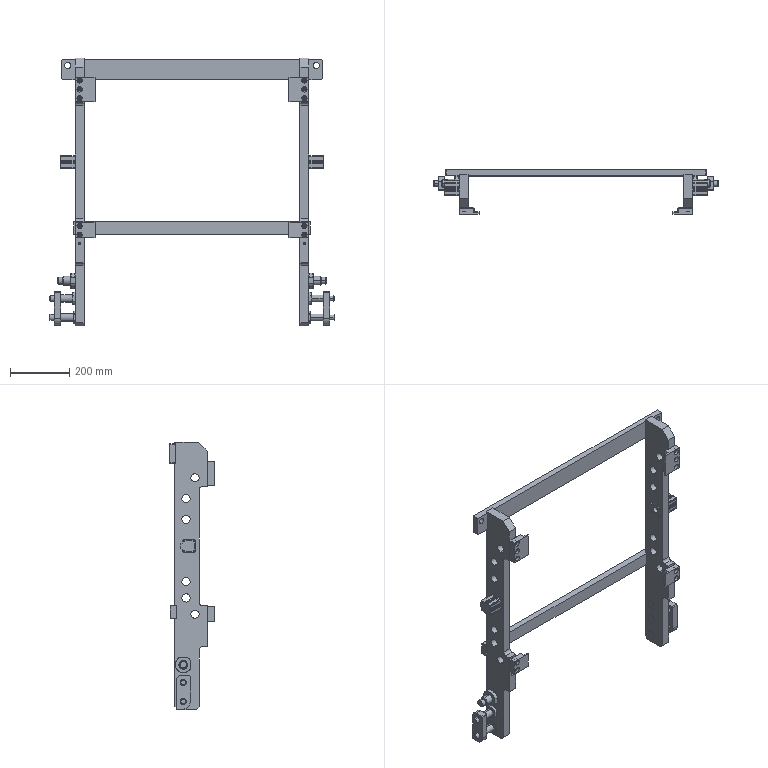Assembly | SolidWorks | mm | 18 component files | 18 solids | 780 faces | box 962 x 150 x 902 mm | volume 7458196 mm3 | plane 354 | cylinder 290 | cone 112 | torus 24 | commonest cylinder face diameters 11 x36 45 x24 28 x24 8.5 x24 32 x24 20 x22 18 x20 6.6 x16
Bill of materials:
EE8-211-_+-_T_w_O(_k) | 1 |  | Long, thin, flat bar with a stepped side profile. One long edge has two raised tabs, and one end is chamfered. A row of through holes runs along the plate; the three holes nearest one end appear to be counterbored or stepped.
EE8-212-_+-_T_w_O(_) | 1 |  | Long, thin, flat bar with a stepped side profile, two tabs on one long edge, a chamfered end, and a row of plain through holes. Looks almost the same as unnamed part except that the end holes have no visible step.
EE8-213-_-_O | 2 |  | Small rectangular block with a step (L-shaped profile) along one edge and three through holes in a line near one side. Some edges are chamfered.
EE8-214-_-_O | 2 |  | Rectangular block with a stepped (rabbeted) side and two through holes near one edge. One end has angled or chamfered faces that form a tapered profile.
FE2-211-_T_w_( | 1 |  | Long, slender rectangular bar. Each end has a short stepped or notched section with one larger hole and two smaller holes.
FE5-217--p_O | 1 |  | Long, slender rectangular bar with a short stepped section at each end, each carrying two holes, one above the other.
FE5-225--a_b | 2 |  | Turned shaft-like part shaped by rotation about one axis. It has a larger cylindrical end, a narrow groove, a flange or collar with flats, and a two-step shaft that narrows toward a chamfered tip.
FE5-226--a_b | 2 |  | Turned shaft-like part similar to unnamed part: a cylindrical end, a groove, a collar with flats, and a stepped shaft with a chamfered tip. The flatted collar section looks longer along the axis.
GL9-204-_v_p_=_v | 2 |  | Box-shaped prism with a constant cross-section along its length. Its profile has cut corners, a T-slot style groove on each of two sides, a notched slot on another side, and four corner through holes running the full length. A wedge-shaped bump runs along one side, and a short cylindrical boss with a chamfer sticks out of one end face.
GL9-236--a_b | 2 |  | Short turned part shaped by rotation about one axis: a cylindrical end, a groove, a small collar, a larger collar with flats, a cylindrical shaft section, and a smaller-diameter tip. Ends are chamfered.
GL9-255--p_O(_k) | 1 |  | Thick rectangular link plate with one fully rounded corner, one small chamfered corner, and two plain through holes along its length.
GL9-257--p_O(_) | 1 |  | Thick rectangular plate with one rounded corner, a chamfered corner, and two through holes. Looks almost the same as unnamed part except that one hole appears to be counterbored or stepped.
Mates:
1. concentric | EE8-211-_+-_T_w_O(_k)-1 face at (15, 81, -524) dir (1, 0, 0) r 16 | FE5-225--a_b-1 face at (102, 81, -524) dir (1, 0, 0) r 16
2. coincident | EE8-211-_+-_T_w_O(_k)-1 face at (7, 81, -524) dir (1, 0, 0) | FE5-225--a_b-1 face at (7, 97, -524) dir (-1, 0, 0)
3. concentric | EE8-211-_+-_T_w_O(_k)-1 face at (15, 81, -460) dir (1, 0, 0) r 16 | FE5-226--a_b-1 face at (100, 81, -460) dir (1, 0, 0) r 16
4. coincident | EE8-211-_+-_T_w_O(_k)-1 face at (7, 81, -460) dir (1, 0, 0) | FE5-226--a_b-1 face at (7, 97, -460) dir (-1, 0, 0)
5. concentric | EE8-211-_+-_T_w_O(_k)-1 face at (15, 81, -400) dir (1, 0, 0) r 16 | GL9-236--a_b-1 face at (-15, 81, -400) dir (-1, 0, 0) r 16
6. coincident | EE8-211-_+-_T_w_O(_k)-1 face at (7, 81, -400) dir (1, 0, 0) | GL9-236--a_b-1 face at (7, 97, -400) dir (-1, 0, 0)
7. parallel | EE8-211-_+-_T_w_O(_k)-1 face at (15, 109.5, 350) dir (0, 1, 0) | GL9-236--a_b-1 face at (73.5, 106.5, -385) dir (0, 1, 0)
8. parallel | EE8-211-_+-_T_w_O(_k)-1 face at (15, 109.5, 350) dir (0, 1, 0) | FE5-226--a_b-1 face at (15, 101.5, -445) dir (0, 1, 0)
9. parallel | EE8-211-_+-_T_w_O(_k)-1 face at (15, 109.5, 350) dir (0, 1, 0) | FE5-225--a_b-1 face at (15, 101.5, -509) dir (0, 1, 0)
10. concentric | FE5-226--a_b-1 face at (100, 81, -460) dir (1, 0, 0) r 10 | GL9-255--p_O(_k)-1 face at (85, 81, -460) dir (-1, 0, 0) r 10
11. concentric | FE5-225--a_b-1 face at (102, 81, -524) dir (1, 0, 0) r 10 | GL9-255--p_O(_k)-1 face at (64, 81, -524) dir (1, 0, 0) r 10
12. coincident | FE5-226--a_b-1 face at (67, 93.5, -460) dir (1, 0, 0) | GL9-255--p_O(_k)-1 face at (67, 81, -460) dir (-1, 0, 0)
13. concentric | EE8-211-_+-_T_w_O(_k)-1 face at (0, 109.5, -210) dir (0, 1, 0) r 5.1 | FE5-217--p_O-1 face at (0, 125.5, -210) dir (0, -1, 0) r 7
14. concentric | EE8-211-_+-_T_w_O(_k)-1 face at (0, 109.5, -235) dir (0, 1, 0) r 5.1 | FE5-217--p_O-1 face at (0, 125.5, -235) dir (0, -1, 0) r 7
15. coincident | EE8-211-_+-_T_w_O(_k)-1 face at (15, 109.5, 350) dir (0, 1, 0) | FE5-217--p_O-1 face at (-15, 109.5, -245) dir (0, -1, 0)
16. concentric | EE8-211-_+-_T_w_O(_k)-1 face at (0, 109.5, 330) dir (0, 1, 0) r 5.1 | FE2-211-_T_w_(-1 face at (0, 126.5, 330) dir (0, -1, 0) r 7
17. concentric | EE8-211-_+-_T_w_O(_k)-1 face at (0, 109.5, 298) dir (0, 1, 0) r 5.1 | FE2-211-_T_w_(-1 face at (0, 126.5, 298) dir (0, -1, 0) r 7
18. coincident | EE8-211-_+-_T_w_O(_k)-1 face at (15, 109.5, 350) dir (0, 1, 0) | FE2-211-_T_w_(-1 face at (-15, 109.5, 278) dir (0, -1, 0)
19. concentric | FE2-211-_T_w_(-1 face at (-758, 126.5, 330) dir (0, -1, 0) r 7 | EE8-212-_+-_T_w_O(_)-1 face at (-758, 109.5, 330) dir (0, 1, 0) r 5.1
20. concentric | FE2-211-_T_w_(-1 face at (-758, 126.5, 298) dir (0, -1, 0) r 7 | EE8-212-_+-_T_w_O(_)-1 face at (-758, 109.5, 298) dir (0, 1, 0) r 5.1
21. coincident | FE2-211-_T_w_(-1 face at (-773, 109.5, 345) dir (0, -1, 0) | EE8-212-_+-_T_w_O(_)-1 face at (-743, 109.5, 350) dir (0, 1, 0)
22. concentric | EE8-212-_+-_T_w_O(_)-1 face at (-743, 81, -400) dir (1, 0, 0) r 16 | GL9-236--a_b-2 face at (-743, 81, -400) dir (1, 0, 0) r 16
23. coincident | EE8-212-_+-_T_w_O(_)-1 face at (-765, 81, -400) dir (-1, 0, 0) | GL9-236--a_b-2 face at (-765, 81, -416) dir (1, 0, 0)
24. concentric | EE8-212-_+-_T_w_O(_)-1 face at (-743, 81, -460) dir (1, 0, 0) r 16 | FE5-226--a_b-2 face at (-858, 81, -460) dir (-1, 0, 0) r 16
25. coincident | EE8-212-_+-_T_w_O(_)-1 face at (-765, 81, -460) dir (-1, 0, 0) | FE5-226--a_b-2 face at (-765, 81, -476) dir (1, 0, 0)
26. concentric | EE8-212-_+-_T_w_O(_)-1 face at (-743, 81, -524) dir (1, 0, 0) r 16 | FE5-225--a_b-2 face at (-860, 81, -524) dir (-1, 0, 0) r 16
27. coincident | EE8-212-_+-_T_w_O(_)-1 face at (-765, 81, -524) dir (-1, 0, 0) | FE5-225--a_b-2 face at (-765, 81, -540) dir (1, 0, 0)
28. parallel | EE8-212-_+-_T_w_O(_)-1 face at (-743, 109.5, 350) dir (0, 1, 0) | GL9-236--a_b-2 face at (-831.5, 106.5, -415) dir (0, 1, 0)
29. parallel | EE8-212-_+-_T_w_O(_)-1 face at (-743, 109.5, 350) dir (0, 1, 0) | FE5-226--a_b-2 face at (-773, 101.5, -475) dir (0, 1, 0)
30. parallel | EE8-212-_+-_T_w_O(_)-1 face at (-743, 109.5, 350) dir (0, 1, 0) | FE5-225--a_b-2 face at (-773, 101.5, -539) dir (0, 1, 0)
31. concentric | FE5-226--a_b-2 face at (-858, 81, -460) dir (-1, 0, 0) r 10 | GL9-257--p_O(_)-1 face at (-843, 81, -460) dir (1, 0, 0) r 10
32. concentric | FE5-225--a_b-2 face at (-860, 81, -524) dir (-1, 0, 0) r 10 | GL9-257--p_O(_)-1 face at (-843, 81, -524) dir (1, 0, 0) r 10
33. coincident | FE5-226--a_b-2 face at (-825, 81, -472.5) dir (-1, 0, 0) | GL9-257--p_O(_)-1 face at (-825, 81, -460) dir (1, 0, 0)
34. concentric | EE8-211-_+-_T_w_O(_k)-1 face at (-15, 78.5, -17) dir (-1, 0, 0) r 3.3 | GL9-204-_v_p_=_v-1 face at (65, 78.5, -17) dir (-1, 0, 0) r 2.6
35. concentric | EE8-211-_+-_T_w_O(_k)-1 face at (-15, 44.5, 17) dir (-1, 0, 0) r 3.3 | GL9-204-_v_p_=_v-1 face at (65, 44.5, 17) dir (-1, 0, 0) r 2.6
36. coincident | EE8-211-_+-_T_w_O(_k)-1 face at (15, 0, 0) dir (1, 0, 0) | GL9-204-_v_p_=_v-1 face at (15, 39.5, 22) dir (-1, 0, 0)
37. concentric | EE8-212-_+-_T_w_O(_)-1 face at (-743, 78.5, -17) dir (1, 0, 0) r 3.3 | GL9-204-_v_p_=_v-2 face at (-823, 78.5, -17) dir (1, 0, 0) r 2.6
38. concentric | EE8-212-_+-_T_w_O(_)-1 face at (-743, 44.5, 17) dir (1, 0, 0) r 3.3 | GL9-204-_v_p_=_v-2 face at (-823, 44.5, 17) dir (1, 0, 0) r 2.6
39. coincident | EE8-212-_+-_T_w_O(_)-1 face at (-773, 0, 0) dir (-1, 0, 0) | GL9-204-_v_p_=_v-2 face at (-773, 39.5, -22) dir (1, 0, 0)
40. concentric | EE8-211-_+-_T_w_O(_k)-1 face at (0, 0, 215) dir (0, -1, 0) r 4.25 | EE8-213-_-_O-1 face at (0, -23.5, 215) dir (0, -1, 0) r 5.5
41. concentric | EE8-211-_+-_T_w_O(_k)-1 face at (0, 0, 275) dir (0, -1, 0) r 4.25 | EE8-213-_-_O-1 face at (0, -23.5, 275) dir (0, -1, 0) r 9
42. coincident | EE8-211-_+-_T_w_O(_k)-1 face at (15, 0, 350) dir (0, -1, 0) | EE8-213-_-_O-1 face at (15, 0, 286) dir (0, 1, 0)
43. concentric | EE8-212-_+-_T_w_O(_)-1 face at (-758, 0, 215) dir (0, -1, 0) r 4.25 | EE8-213-_-_O-2 face at (-758, -23.5, 215) dir (0, -1, 0) r 5.5
44. concentric | EE8-212-_+-_T_w_O(_)-1 face at (-758, 0, 275) dir (0, -1, 0) r 4.25 | EE8-213-_-_O-2 face at (-758, -23.5, 275) dir (0, -1, 0) r 9
45. coincident | EE8-212-_+-_T_w_O(_)-1 face at (-743, 0, 350) dir (0, -1, 0) | EE8-213-_-_O-2 face at (-773, 0, 204) dir (0, 1, 0)
46. concentric | EE8-211-_+-_T_w_O(_k)-1 face at (0, 0, -245) dir (0, -1, 0) r 4.25 | EE8-214-_-_O-2 face at (0, -23.5, -245) dir (0, -1, 0) r 5.5
47. concentric | EE8-211-_+-_T_w_O(_k)-1 face at (0, 0, -215) dir (0, -1, 0) r 4.25 | EE8-214-_-_O-2 face at (0, -23.5, -215) dir (0, -1, 0) r 9
48. coincident | EE8-211-_+-_T_w_O(_k)-1 face at (15, 0, 350) dir (0, -1, 0) | EE8-214-_-_O-2 face at (15, 0, -204) dir (0, 1, 0)
49. concentric | EE8-212-_+-_T_w_O(_)-1 face at (-758, 0, -215) dir (0, -1, 0) r 4.25 | EE8-214-_-_O-1 face at (-758, -23.5, -215) dir (0, -1, 0) r 5.5
50. concentric | EE8-212-_+-_T_w_O(_)-1 face at (-758, 0, -245) dir (0, -1, 0) r 4.25 | EE8-214-_-_O-1 face at (-758, -23.5, -245) dir (0, -1, 0) r 9
51. coincident | EE8-212-_+-_T_w_O(_)-1 face at (-743, 0, 350) dir (0, -1, 0) | EE8-214-_-_O-1 face at (-773, 0, -256) dir (0, 1, 0)